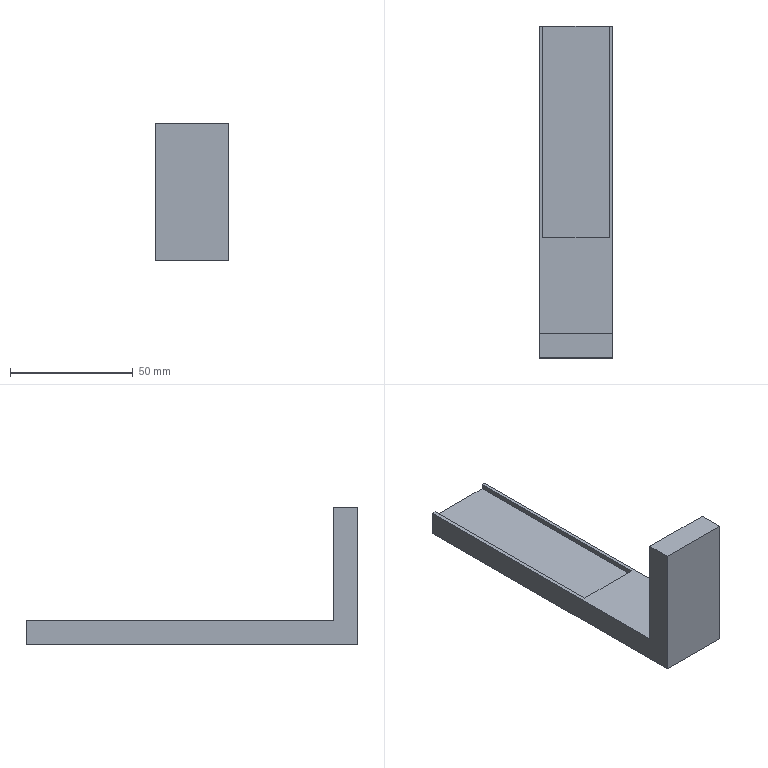Component | SolidWorks | Gripper-2024-3-4-05-1 | 1 solid | 12 faces | box 30 x 135 x 56 mm | volume 49656 mm3 | plane 12 | material AL6061
build123d program:
from build123d import *

# Parameters (mm, degrees)
BOSS_EXTRUDE1_DEPTH = 30
SKETCH2_W           = 172
SKETCH2_H           = 27
CUT_EXTRUDE1_DEPTH  = 2


with BuildPart() as part:
    # Sketch1 → Boss-Extrude1 (new body)
    with BuildSketch(Plane.XY):
        Polygon((0, 0), (10, 0), (10, 46), (135, 46), (135, 56), (10, 56), (0, 56), align=None)
    extrude(amount=BOSS_EXTRUDE1_DEPTH)

    # Sketch2 → Cut-Extrude1 (cut)
    with BuildSketch(Plane.XZ.offset(-46)):
        with Locations((135, 15)):
            Rectangle(SKETCH2_W, SKETCH2_H)
    extrude(amount=-CUT_EXTRUDE1_DEPTH, mode=Mode.SUBTRACT)


solid = part.part

# Placed as in the assembly
solid = solid.moved(Location((-85.094, -141.769, 330), (-90, -90, 0)))
STEP:
#1=CARTESIAN_POINT('',(-3.35,-5.581,10.787));
#2=VERTEX_POINT('',#1);
#3=CARTESIAN_POINT('',(-3.35,-5.581,12.992));
#4=VERTEX_POINT('',#3);
#5=CARTESIAN_POINT('',(-3.35,-5.581,12.992));
#6=DIRECTION('',(-0.,-0.,1.));
#7=VECTOR('',#6,39.37);
#8=LINE('',#5,#7);
#9=EDGE_CURVE('',#2,#4,#8,.T.);
#10=ORIENTED_EDGE('',*,*,#9,.T.);
#11=CARTESIAN_POINT('',(-4.531,-5.581,12.992));
#12=VERTEX_POINT('',#11);
#13=CARTESIAN_POINT('',(-4.531,-5.581,12.992));
#14=DIRECTION('',(1.,0.,0.));
#15=VECTOR('',#14,39.37);
#16=LINE('',#13,#15);
#17=EDGE_CURVE('',#12,#4,#16,.T.);
#18=ORIENTED_EDGE('',*,*,#17,.F.);
#19=CARTESIAN_POINT('',(-4.531,-5.581,10.787));
#20=VERTEX_POINT('',#19);
#21=CARTESIAN_POINT('',(-4.531,-5.581,12.992));
#22=DIRECTION('',(-0.,-0.,1.));
#23=VECTOR('',#22,39.37);
#24=LINE('',#21,#23);
#25=EDGE_CURVE('',#20,#12,#24,.T.);
#26=ORIENTED_EDGE('',*,*,#25,.F.);
#27=CARTESIAN_POINT('',(-4.531,-5.581,10.787));
#28=DIRECTION('',(1.,0.,0.));
#29=VECTOR('',#28,39.37);
#30=LINE('',#27,#29);
#31=EDGE_CURVE('',#20,#2,#30,.T.);
#32=ORIENTED_EDGE('',*,*,#31,.T.);
#33=EDGE_LOOP('',(#10,#18,#26,#32));
#34=FACE_OUTER_BOUND('',#33,.T.);
#35=CARTESIAN_POINT('',(-4.531,-5.581,12.992));
#36=DIRECTION('',(-0.,1.,0.));
#37=DIRECTION('',(1.,0.,0.));
#38=AXIS2_PLACEMENT_3D('',#35,#36,#37);
#39=PLANE('',#38);
#40=ADVANCED_FACE('',(#34),#39,.F.);
#41=CARTESIAN_POINT('',(-3.35,-5.188,12.992));
#42=VERTEX_POINT('',#41);
#43=CARTESIAN_POINT('',(-3.35,-5.581,12.992));
#44=DIRECTION('',(0.,1.,0.));
#45=VECTOR('',#44,39.37);
#46=LINE('',#43,#45);
#47=EDGE_CURVE('',#4,#42,#46,.T.);
#48=ORIENTED_EDGE('',*,*,#47,.T.);
#49=CARTESIAN_POINT('',(-4.531,-5.188,12.992));
#50=VERTEX_POINT('',#49);
#51=CARTESIAN_POINT('',(-4.531,-5.188,12.992));
#52=DIRECTION('',(1.,0.,0.));
#53=VECTOR('',#52,39.37);
#54=LINE('',#51,#53);
#55=EDGE_CURVE('',#50,#42,#54,.T.);
#56=ORIENTED_EDGE('',*,*,#55,.F.);
#57=CARTESIAN_POINT('',(-4.531,-5.581,12.992));
#58=DIRECTION('',(0.,1.,0.));
#59=VECTOR('',#58,39.37);
#60=LINE('',#57,#59);
#61=EDGE_CURVE('',#12,#50,#60,.T.);
#62=ORIENTED_EDGE('',*,*,#61,.F.);
#63=ORIENTED_EDGE('',*,*,#17,.T.);
#64=EDGE_LOOP('',(#48,#56,#62,#63));
#65=FACE_OUTER_BOUND('',#64,.T.);
#66=CARTESIAN_POINT('',(-4.531,-5.581,12.992));
#67=DIRECTION('',(0.,0.,-1.));
#68=DIRECTION('',(-1.,-0.,-0.));
#69=AXIS2_PLACEMENT_3D('',#66,#67,#68);
#70=PLANE('',#69);
#71=ADVANCED_FACE('',(#65),#70,.F.);
#72=CARTESIAN_POINT('',(-3.35,-5.188,11.181));
#73=VERTEX_POINT('',#72);
#74=CARTESIAN_POINT('',(-3.35,-5.188,12.992));
#75=DIRECTION('',(0.,0.,-1.));
#76=VECTOR('',#75,39.37);
#77=LINE('',#74,#76);
#78=EDGE_CURVE('',#42,#73,#77,.T.);
#79=ORIENTED_EDGE('',*,*,#78,.T.);
#80=CARTESIAN_POINT('',(-4.531,-5.188,11.181));
#81=VERTEX_POINT('',#80);
#82=CARTESIAN_POINT('',(-4.531,-5.188,11.181));
#83=DIRECTION('',(1.,0.,0.));
#84=VECTOR('',#83,39.37);
#85=LINE('',#82,#84);
#86=EDGE_CURVE('',#81,#73,#85,.T.);
#87=ORIENTED_EDGE('',*,*,#86,.F.);
#88=CARTESIAN_POINT('',(-4.531,-5.188,12.992));
#89=DIRECTION('',(0.,0.,-1.));
#90=VECTOR('',#89,39.37);
#91=LINE('',#88,#90);
#92=EDGE_CURVE('',#50,#81,#91,.T.);
#93=ORIENTED_EDGE('',*,*,#92,.F.);
#94=ORIENTED_EDGE('',*,*,#55,.T.);
#95=EDGE_LOOP('',(#79,#87,#93,#94));
#96=FACE_OUTER_BOUND('',#95,.T.);
#97=CARTESIAN_POINT('',(-4.531,-5.188,12.992));
#98=DIRECTION('',(0.,-1.,-0.));
#99=DIRECTION('',(-1.,-0.,-0.));
#100=AXIS2_PLACEMENT_3D('',#97,#98,#99);
#101=PLANE('',#100);
#102=ADVANCED_FACE('',(#96),#101,.F.);
#103=CARTESIAN_POINT('',(-4.472,-3.652,11.181));
#104=VERTEX_POINT('',#103);
#105=CARTESIAN_POINT('',(-3.409,-3.652,11.181));
#106=VERTEX_POINT('',#105);
#107=CARTESIAN_POINT('',(-4.472,-3.652,11.181));
#108=DIRECTION('',(1.,0.,0.));
#109=VECTOR('',#108,39.37);
#110=LINE('',#107,#109);
#111=EDGE_CURVE('',#104,#106,#110,.T.);
#112=ORIENTED_EDGE('',*,*,#111,.F.);
#113=CARTESIAN_POINT('',(-4.472,-0.2665,11.181));
#114=VERTEX_POINT('',#113);
#115=CARTESIAN_POINT('',(-4.472,3.119,11.181));
#116=DIRECTION('',(0.,-1.,-0.));
#117=VECTOR('',#116,39.37);
#118=LINE('',#115,#117);
#119=EDGE_CURVE('',#114,#104,#118,.T.);
#120=ORIENTED_EDGE('',*,*,#119,.F.);
#121=CARTESIAN_POINT('',(-4.531,-0.2665,11.181));
#122=VERTEX_POINT('',#121);
#123=CARTESIAN_POINT('',(-4.531,-0.2665,11.181));
#124=DIRECTION('',(1.,0.,0.));
#125=VECTOR('',#124,39.37);
#126=LINE('',#123,#125);
#127=EDGE_CURVE('',#122,#114,#126,.T.);
#128=ORIENTED_EDGE('',*,*,#127,.F.);
#129=CARTESIAN_POINT('',(-4.531,-5.188,11.181));
#130=DIRECTION('',(0.,1.,0.));
#131=VECTOR('',#130,39.37);
#132=LINE('',#129,#131);
#133=EDGE_CURVE('',#81,#122,#132,.T.);
#134=ORIENTED_EDGE('',*,*,#133,.F.);
#135=ORIENTED_EDGE('',*,*,#86,.T.);
#136=CARTESIAN_POINT('',(-3.35,-0.2665,11.181));
#137=VERTEX_POINT('',#136);
#138=CARTESIAN_POINT('',(-3.35,-5.188,11.181));
#139=DIRECTION('',(0.,1.,0.));
#140=VECTOR('',#139,39.37);
#141=LINE('',#138,#140);
#142=EDGE_CURVE('',#73,#137,#141,.T.);
#143=ORIENTED_EDGE('',*,*,#142,.T.);
#144=CARTESIAN_POINT('',(-3.409,-0.2665,11.181));
#145=VERTEX_POINT('',#144);
#146=CARTESIAN_POINT('',(-4.531,-0.2665,11.181));
#147=DIRECTION('',(1.,0.,0.));
#148=VECTOR('',#147,39.37);
#149=LINE('',#146,#148);
#150=EDGE_CURVE('',#145,#137,#149,.T.);
#151=ORIENTED_EDGE('',*,*,#150,.F.);
#152=CARTESIAN_POINT('',(-3.409,3.119,11.181));
#153=DIRECTION('',(-0.,1.,0.));
#154=VECTOR('',#153,39.37);
#155=LINE('',#152,#154);
#156=EDGE_CURVE('',#106,#145,#155,.T.);
#157=ORIENTED_EDGE('',*,*,#156,.F.);
#158=EDGE_LOOP('',(#112,#120,#128,#134,#135,#143,#151,#157));
#159=FACE_OUTER_BOUND('',#158,.T.);
#160=CARTESIAN_POINT('',(-4.531,-5.188,11.181));
#161=DIRECTION('',(0.,0.,-1.));
#162=DIRECTION('',(-1.,-0.,-0.));
#163=AXIS2_PLACEMENT_3D('',#160,#161,#162);
#164=PLANE('',#163);
#165=ADVANCED_FACE('',(#159),#164,.F.);
#166=ORIENTED_EDGE('',*,*,#127,.T.);
#167=CARTESIAN_POINT('',(-4.472,-0.2665,11.102));
#168=VERTEX_POINT('',#167);
#169=CARTESIAN_POINT('',(-4.472,-0.2665,10.787));
#170=DIRECTION('',(0.,0.,-1.));
#171=VECTOR('',#170,39.37);
#172=LINE('',#169,#171);
#173=EDGE_CURVE('',#114,#168,#172,.T.);
#174=ORIENTED_EDGE('',*,*,#173,.T.);
#175=CARTESIAN_POINT('',(-3.409,-0.2665,11.102));
#176=VERTEX_POINT('',#175);
#177=CARTESIAN_POINT('',(-4.531,-0.2665,11.102));
#178=DIRECTION('',(1.,0.,0.));
#179=VECTOR('',#178,39.37);
#180=LINE('',#177,#179);
#181=EDGE_CURVE('',#168,#176,#180,.T.);
#182=ORIENTED_EDGE('',*,*,#181,.T.);
#183=CARTESIAN_POINT('',(-3.409,-0.2665,10.787));
#184=DIRECTION('',(-0.,-0.,1.));
#185=VECTOR('',#184,39.37);
#186=LINE('',#183,#185);
#187=EDGE_CURVE('',#176,#145,#186,.T.);
#188=ORIENTED_EDGE('',*,*,#187,.T.);
#189=ORIENTED_EDGE('',*,*,#150,.T.);
#190=CARTESIAN_POINT('',(-3.35,-0.2665,10.787));
#191=VERTEX_POINT('',#190);
#192=CARTESIAN_POINT('',(-3.35,-0.2665,10.787));
#193=DIRECTION('',(0.,0.,-1.));
#194=VECTOR('',#193,39.37);
#195=LINE('',#192,#194);
#196=EDGE_CURVE('',#137,#191,#195,.T.);
#197=ORIENTED_EDGE('',*,*,#196,.T.);
#198=CARTESIAN_POINT('',(-4.531,-0.2665,10.787));
#199=VERTEX_POINT('',#198);
#200=CARTESIAN_POINT('',(-4.531,-0.2665,10.787));
#201=DIRECTION('',(1.,0.,0.));
#202=VECTOR('',#201,39.37);
#203=LINE('',#200,#202);
#204=EDGE_CURVE('',#199,#191,#203,.T.);
#205=ORIENTED_EDGE('',*,*,#204,.F.);
#206=CARTESIAN_POINT('',(-4.531,-0.2665,10.787));
#207=DIRECTION('',(0.,0.,-1.));
#208=VECTOR('',#207,39.37);
#209=LINE('',#206,#208);
#210=EDGE_CURVE('',#122,#199,#209,.T.);
#211=ORIENTED_EDGE('',*,*,#210,.F.);
#212=EDGE_LOOP('',(#166,#174,#182,#188,#189,#197,#205,#211));
#213=FACE_OUTER_BOUND('',#212,.T.);
#214=CARTESIAN_POINT('',(-4.531,-0.2665,10.787));
#215=DIRECTION('',(0.,-1.,-0.));
#216=DIRECTION('',(-1.,-0.,-0.));
#217=AXIS2_PLACEMENT_3D('',#214,#215,#216);
#218=PLANE('',#217);
#219=ADVANCED_FACE('',(#213),#218,.F.);
#220=CARTESIAN_POINT('',(-3.35,-5.581,10.787));
#221=DIRECTION('',(-0.,-1.,-0.));
#222=VECTOR('',#221,39.37);
#223=LINE('',#220,#222);
#224=EDGE_CURVE('',#191,#2,#223,.T.);
#225=ORIENTED_EDGE('',*,*,#224,.T.);
#226=ORIENTED_EDGE('',*,*,#31,.F.);
#227=CARTESIAN_POINT('',(-4.531,-5.188,10.787));
#228=DIRECTION('',(-0.,-1.,-0.));
#229=VECTOR('',#228,39.37);
#230=LINE('',#227,#229);
#231=EDGE_CURVE('',#199,#20,#230,.T.);
#232=ORIENTED_EDGE('',*,*,#231,.F.);
#233=ORIENTED_EDGE('',*,*,#204,.T.);
#234=EDGE_LOOP('',(#225,#226,#232,#233));
#235=FACE_OUTER_BOUND('',#234,.T.);
#236=CARTESIAN_POINT('',(-4.531,-5.581,10.787));
#237=DIRECTION('',(-0.,-0.,1.));
#238=DIRECTION('',(1.,0.,0.));
#239=AXIS2_PLACEMENT_3D('',#236,#237,#238);
#240=PLANE('',#239);
#241=ADVANCED_FACE('',(#235),#240,.F.);
#242=ORIENTED_EDGE('',*,*,#25,.T.);
#243=ORIENTED_EDGE('',*,*,#61,.T.);
#244=ORIENTED_EDGE('',*,*,#92,.T.);
#245=ORIENTED_EDGE('',*,*,#133,.T.);
#246=ORIENTED_EDGE('',*,*,#210,.T.);
#247=ORIENTED_EDGE('',*,*,#231,.T.);
#248=EDGE_LOOP('',(#242,#243,#244,#245,#246,#247));
#249=FACE_OUTER_BOUND('',#248,.T.);
#250=CARTESIAN_POINT('',(-4.531,-5.581,12.992));
#251=DIRECTION('',(1.,-0.,0.));
#252=DIRECTION('',(-0.,-1.,-0.));
#253=AXIS2_PLACEMENT_3D('',#250,#251,#252);
#254=PLANE('',#253);
#255=ADVANCED_FACE('',(#249),#254,.F.);
#256=ORIENTED_EDGE('',*,*,#9,.F.);
#257=ORIENTED_EDGE('',*,*,#224,.F.);
#258=ORIENTED_EDGE('',*,*,#196,.F.);
#259=ORIENTED_EDGE('',*,*,#142,.F.);
#260=ORIENTED_EDGE('',*,*,#78,.F.);
#261=ORIENTED_EDGE('',*,*,#47,.F.);
#262=EDGE_LOOP('',(#256,#257,#258,#259,#260,#261));
#263=FACE_OUTER_BOUND('',#262,.T.);
#264=CARTESIAN_POINT('',(-3.35,-5.581,12.992));
#265=DIRECTION('',(1.,-0.,0.));
#266=DIRECTION('',(-0.,-1.,-0.));
#267=AXIS2_PLACEMENT_3D('',#264,#265,#266);
#268=PLANE('',#267);
#269=ADVANCED_FACE('',(#263),#268,.T.);
#270=ORIENTED_EDGE('',*,*,#119,.T.);
#271=CARTESIAN_POINT('',(-4.472,-3.652,11.102));
#272=VERTEX_POINT('',#271);
#273=CARTESIAN_POINT('',(-4.472,-3.652,11.102));
#274=DIRECTION('',(-0.,-0.,1.));
#275=VECTOR('',#274,39.37);
#276=LINE('',#273,#275);
#277=EDGE_CURVE('',#272,#104,#276,.T.);
#278=ORIENTED_EDGE('',*,*,#277,.F.);
#279=CARTESIAN_POINT('',(-4.472,3.119,11.102));
#280=DIRECTION('',(0.,-1.,-0.));
#281=VECTOR('',#280,39.37);
#282=LINE('',#279,#281);
#283=EDGE_CURVE('',#168,#272,#282,.T.);
#284=ORIENTED_EDGE('',*,*,#283,.F.);
#285=ORIENTED_EDGE('',*,*,#173,.F.);
#286=EDGE_LOOP('',(#270,#278,#284,#285));
#287=FACE_OUTER_BOUND('',#286,.T.);
#288=CARTESIAN_POINT('',(-4.472,3.119,11.102));
#289=DIRECTION('',(-1.,-0.,-0.));
#290=DIRECTION('',(-0.,1.,0.));
#291=AXIS2_PLACEMENT_3D('',#288,#289,#290);
#292=PLANE('',#291);
#293=ADVANCED_FACE('',(#287),#292,.F.);
#294=CARTESIAN_POINT('',(-3.409,-3.652,11.102));
#295=VERTEX_POINT('',#294);
#296=CARTESIAN_POINT('',(-3.409,3.119,11.102));
#297=DIRECTION('',(-0.,1.,0.));
#298=VECTOR('',#297,39.37);
#299=LINE('',#296,#298);
#300=EDGE_CURVE('',#295,#176,#299,.T.);
#301=ORIENTED_EDGE('',*,*,#300,.F.);
#302=CARTESIAN_POINT('',(-3.409,-3.652,11.102));
#303=DIRECTION('',(-0.,-0.,1.));
#304=VECTOR('',#303,39.37);
#305=LINE('',#302,#304);
#306=EDGE_CURVE('',#295,#106,#305,.T.);
#307=ORIENTED_EDGE('',*,*,#306,.T.);
#308=ORIENTED_EDGE('',*,*,#156,.T.);
#309=ORIENTED_EDGE('',*,*,#187,.F.);
#310=EDGE_LOOP('',(#301,#307,#308,#309));
#311=FACE_OUTER_BOUND('',#310,.T.);
#312=CARTESIAN_POINT('',(-3.409,3.119,11.102));
#313=DIRECTION('',(1.,0.,0.));
#314=DIRECTION('',(0.,-1.,-0.));
#315=AXIS2_PLACEMENT_3D('',#312,#313,#314);
#316=PLANE('',#315);
#317=ADVANCED_FACE('',(#311),#316,.F.);
#318=ORIENTED_EDGE('',*,*,#283,.T.);
#319=CARTESIAN_POINT('',(-4.472,-3.652,11.102));
#320=DIRECTION('',(1.,0.,0.));
#321=VECTOR('',#320,39.37);
#322=LINE('',#319,#321);
#323=EDGE_CURVE('',#272,#295,#322,.T.);
#324=ORIENTED_EDGE('',*,*,#323,.T.);
#325=ORIENTED_EDGE('',*,*,#300,.T.);
#326=ORIENTED_EDGE('',*,*,#181,.F.);
#327=EDGE_LOOP('',(#318,#324,#325,#326));
#328=FACE_OUTER_BOUND('',#327,.T.);
#329=CARTESIAN_POINT('',(-3.35,-5.581,11.102));
#330=DIRECTION('',(0.,0.,-1.));
#331=DIRECTION('',(-1.,-0.,-0.));
#332=AXIS2_PLACEMENT_3D('',#329,#330,#331);
#333=PLANE('',#332);
#334=ADVANCED_FACE('',(#328),#333,.F.);
#335=ORIENTED_EDGE('',*,*,#111,.T.);
#336=ORIENTED_EDGE('',*,*,#306,.F.);
#337=ORIENTED_EDGE('',*,*,#323,.F.);
#338=ORIENTED_EDGE('',*,*,#277,.T.);
#339=EDGE_LOOP('',(#335,#336,#337,#338));
#340=FACE_OUTER_BOUND('',#339,.T.);
#341=CARTESIAN_POINT('',(-4.472,-3.652,11.102));
#342=DIRECTION('',(0.,-1.,-0.));
#343=DIRECTION('',(-1.,-0.,-0.));
#344=AXIS2_PLACEMENT_3D('',#341,#342,#343);
#345=PLANE('',#344);
#346=ADVANCED_FACE('',(#340),#345,.F.);
#347=CLOSED_SHELL('',(#40,#71,#102,#165,#219,#241,#255,#269,#293,#317,#334,#346));
#348=MANIFOLD_SOLID_BREP('',#347);
#349=CARTESIAN_POINT('',(0.,0.,0.));
#350=DIRECTION('',(0.,0.,1.));
#351=DIRECTION('',(1.,0.,0.));
#352=AXIS2_PLACEMENT_3D('',#349,#350,#351);
#353=(LENGTH_UNIT()NAMED_UNIT(*)SI_UNIT($,.METRE.));
#354=LENGTH_MEASURE_WITH_UNIT(LENGTH_MEASURE(0.0254),#353);
#355=DIMENSIONAL_EXPONENTS(1.,0.,0.,0.,0.,0.,0.);
#356=(CONVERSION_BASED_UNIT('',#354)LENGTH_UNIT()NAMED_UNIT(#355));
#357=UNCERTAINTY_MEASURE_WITH_UNIT(LENGTH_MEASURE(0.00001),#356,'','');
#358=(NAMED_UNIT(*)PLANE_ANGLE_UNIT()SI_UNIT($,.RADIAN.));
#359=(NAMED_UNIT(*)SI_UNIT($,.STERADIAN.)SOLID_ANGLE_UNIT());
#360=(GEOMETRIC_REPRESENTATION_CONTEXT(3)GLOBAL_UNCERTAINTY_ASSIGNED_CONTEXT((#357))GLOBAL_UNIT_ASSIGNED_CONTEXT((#356,#358,#359))REPRESENTATION_CONTEXT('',''));
#361=ADVANCED_BREP_SHAPE_REPRESENTATION('',(#348,#352),#360);
#362=COLOUR_RGB('',0.7922,0.8196,0.9333);
#363=FILL_AREA_STYLE_COLOUR('',#362);
#364=FILL_AREA_STYLE('',(#363));
#365=SURFACE_STYLE_FILL_AREA(#364);
#366=SURFACE_SIDE_STYLE('',(#365));
#367=SURFACE_STYLE_USAGE(.BOTH.,#366);
#368=PRESENTATION_STYLE_ASSIGNMENT((#367));
#369=STYLED_ITEM('',(#368),#348);
#370=(LENGTH_UNIT()NAMED_UNIT(*)SI_UNIT($,.METRE.));
#371=LENGTH_MEASURE_WITH_UNIT(LENGTH_MEASURE(0.0254),#370);
#372=DIMENSIONAL_EXPONENTS(1.,0.,0.,0.,0.,0.,0.);
#373=(CONVERSION_BASED_UNIT('',#371)LENGTH_UNIT()NAMED_UNIT(#372));
#374=UNCERTAINTY_MEASURE_WITH_UNIT(LENGTH_MEASURE(0.00001),#373,'','');
#375=(NAMED_UNIT(*)PLANE_ANGLE_UNIT()SI_UNIT($,.RADIAN.));
#376=(NAMED_UNIT(*)SI_UNIT($,.STERADIAN.)SOLID_ANGLE_UNIT());
#377=(GEOMETRIC_REPRESENTATION_CONTEXT(3)GLOBAL_UNCERTAINTY_ASSIGNED_CONTEXT((#374))GLOBAL_UNIT_ASSIGNED_CONTEXT((#373,#375,#376))REPRESENTATION_CONTEXT('',''));
#378=MECHANICAL_DESIGN_GEOMETRIC_PRESENTATION_REPRESENTATION('',(#369),#377);
#379=PRESENTATION_LAYER_ASSIGNMENT('','',(#369));